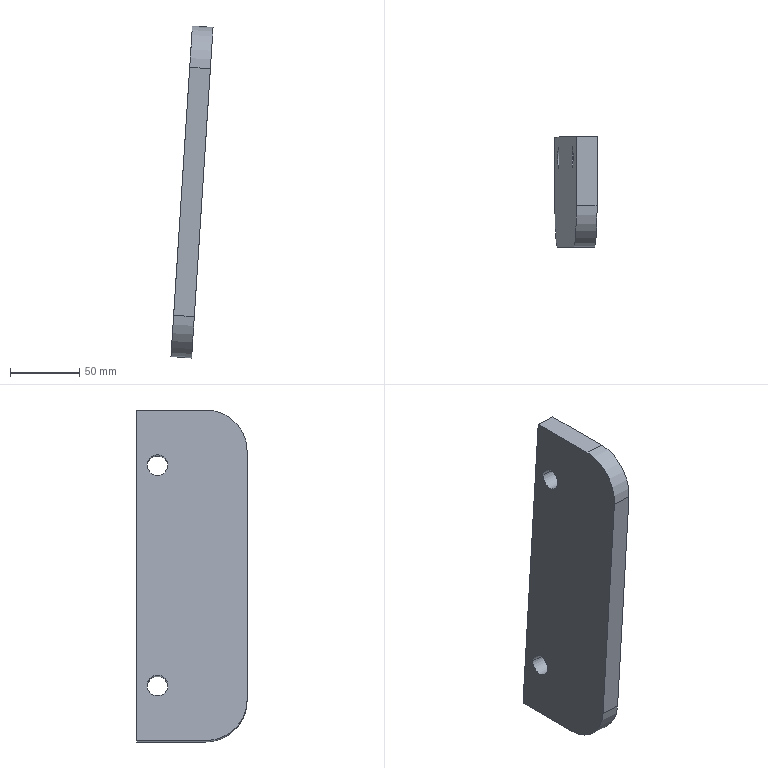Component | SolidWorks | Baffle-2 | 1 solid | 12 faces | box 30.51 x 80 x 240.47 mm | volume 276904 mm3 | cylinder 6 | plane 6 | commonest cylinder face diameters 15 x4 60 x2
build123d program:
from build123d import *

# Parameters (mm, degrees)
BOSS_EXTRUDE1_DEPTH     = 15
CUT_EXTRUDE1_DEPTH      = 697.32
CUT_EXTRUDE1_DEPTH_BACK = 697.32
SKETCH2_R               = 7.5


with BuildPart() as part:
    # Sketch1 → Boss-Extrude1 (new body)
    with BuildSketch(Plane.XY):
        with BuildLine():
            Line((0, 691.546), (50, 691.546))
            ThreePointArc((50, 691.546), (71.213, 682.759), (80, 661.546))
            Line((80, 661.546), (80, 481.546))
            ThreePointArc((80, 481.546), (71.213, 460.333), (50, 451.546))
            Line((50, 451.546), (0, 451.546))
            Line((0, 451.546), (0, 691.546))
        make_face()
    extrude(amount=BOSS_EXTRUDE1_DEPTH)

    # Sketch2 → Cut-Extrude1 (cut, two sides: drawn at the far end of the back side and taken through both)
    with BuildSketch(Plane.XY.offset(15).offset(-CUT_EXTRUDE1_DEPTH_BACK)):
        with Locations((15, 491.546)):
            Circle(SKETCH2_R)
        with Locations((15, 651.546)):
            Circle(SKETCH2_R)
    extrude(amount=CUT_EXTRUDE1_DEPTH + CUT_EXTRUDE1_DEPTH_BACK, mode=Mode.SUBTRACT)


solid = part.part

# Placed as in the assembly
solid = solid.moved(Location((446.042, -801, 253.969), (-180, 86.288, 90)))
STEP:
#1=COLOUR_RGB('',0.7922,0.8196,0.9333);
#2=FILL_AREA_STYLE_COLOUR('',#1);
#3=FILL_AREA_STYLE('',(#2));
#4=SURFACE_STYLE_FILL_AREA(#3);
#5=SURFACE_SIDE_STYLE('',(#4));
#6=SURFACE_STYLE_USAGE(.BOTH.,#5);
#7=PRESENTATION_STYLE_ASSIGNMENT((#6));
#8=CARTESIAN_POINT('',(16.308,-31.831,-9.313));
#9=VERTEX_POINT('',#8);
#10=CARTESIAN_POINT('',(16.308,-32.421,-9.313));
#11=VERTEX_POINT('',#10);
#12=CARTESIAN_POINT('',(16.308,-32.126,-9.313));
#13=DIRECTION('',(0.9979,0.,-0.06474));
#14=DIRECTION('',(0.,-1.,0.));
#15=AXIS2_PLACEMENT_3D('',#12,#13,#14);
#16=CIRCLE('',#15,0.2953);
#17=EDGE_CURVE('',#9,#11,#16,.T.);
#18=ORIENTED_EDGE('',*,*,#17,.F.);
#19=CARTESIAN_POINT('',(16.897,-31.831,-9.351));
#20=VERTEX_POINT('',#19);
#21=CARTESIAN_POINT('',(16.308,-31.831,-9.313));
#22=DIRECTION('',(0.9979,0.,-0.06474));
#23=VECTOR('',#22,39.37);
#24=LINE('',#21,#23);
#25=EDGE_CURVE('',#9,#20,#24,.T.);
#26=ORIENTED_EDGE('',*,*,#25,.T.);
#27=CARTESIAN_POINT('',(16.897,-32.421,-9.351));
#28=VERTEX_POINT('',#27);
#29=CARTESIAN_POINT('',(16.897,-32.126,-9.351));
#30=DIRECTION('',(0.9979,0.,-0.06474));
#31=DIRECTION('',(0.,-1.,0.));
#32=AXIS2_PLACEMENT_3D('',#29,#30,#31);
#33=CIRCLE('',#32,0.2953);
#34=EDGE_CURVE('',#20,#28,#33,.T.);
#35=ORIENTED_EDGE('',*,*,#34,.T.);
#36=CARTESIAN_POINT('',(16.308,-32.421,-9.313));
#37=DIRECTION('',(0.9979,0.,-0.06474));
#38=VECTOR('',#37,39.37);
#39=LINE('',#36,#38);
#40=EDGE_CURVE('',#11,#28,#39,.T.);
#41=ORIENTED_EDGE('',*,*,#40,.F.);
#42=EDGE_LOOP('',(#18,#26,#35,#41));
#43=FACE_OUTER_BOUND('',#42,.T.);
#44=CARTESIAN_POINT('',(16.308,-32.126,-9.313));
#45=DIRECTION('',(0.9979,0.,-0.06474));
#46=DIRECTION('',(0.,-1.,0.));
#47=AXIS2_PLACEMENT_3D('',#44,#45,#46);
#48=CYLINDRICAL_SURFACE('',#47,0.2953);
#49=ADVANCED_FACE('',(#43),#48,.F.);
#50=CARTESIAN_POINT('',(15.9,-31.831,-15.599));
#51=VERTEX_POINT('',#50);
#52=CARTESIAN_POINT('',(15.9,-32.421,-15.599));
#53=VERTEX_POINT('',#52);
#54=CARTESIAN_POINT('',(15.9,-32.126,-15.599));
#55=DIRECTION('',(0.9979,0.,-0.06474));
#56=DIRECTION('',(0.,1.,0.));
#57=AXIS2_PLACEMENT_3D('',#54,#55,#56);
#58=CIRCLE('',#57,0.2953);
#59=EDGE_CURVE('',#51,#53,#58,.T.);
#60=ORIENTED_EDGE('',*,*,#59,.F.);
#61=CARTESIAN_POINT('',(16.489,-31.831,-15.637));
#62=VERTEX_POINT('',#61);
#63=CARTESIAN_POINT('',(15.9,-31.831,-15.599));
#64=DIRECTION('',(0.9979,0.,-0.06474));
#65=VECTOR('',#64,39.37);
#66=LINE('',#63,#65);
#67=EDGE_CURVE('',#51,#62,#66,.T.);
#68=ORIENTED_EDGE('',*,*,#67,.T.);
#69=CARTESIAN_POINT('',(16.489,-32.421,-15.637));
#70=VERTEX_POINT('',#69);
#71=CARTESIAN_POINT('',(16.489,-32.126,-15.637));
#72=DIRECTION('',(0.9979,0.,-0.06474));
#73=DIRECTION('',(0.,-1.,0.));
#74=AXIS2_PLACEMENT_3D('',#71,#72,#73);
#75=CIRCLE('',#74,0.2953);
#76=EDGE_CURVE('',#62,#70,#75,.T.);
#77=ORIENTED_EDGE('',*,*,#76,.T.);
#78=CARTESIAN_POINT('',(15.9,-32.421,-15.599));
#79=DIRECTION('',(0.9979,0.,-0.06474));
#80=VECTOR('',#79,39.37);
#81=LINE('',#78,#80);
#82=EDGE_CURVE('',#53,#70,#81,.T.);
#83=ORIENTED_EDGE('',*,*,#82,.F.);
#84=EDGE_LOOP('',(#60,#68,#77,#83));
#85=FACE_OUTER_BOUND('',#84,.T.);
#86=CARTESIAN_POINT('',(15.9,-32.126,-15.599));
#87=DIRECTION('',(0.9979,0.,-0.06474));
#88=DIRECTION('',(0.,-1.,0.));
#89=AXIS2_PLACEMENT_3D('',#86,#87,#88);
#90=CYLINDRICAL_SURFACE('',#89,0.2953);
#91=ADVANCED_FACE('',(#85),#90,.F.);
#92=CARTESIAN_POINT('',(15.798,-31.535,-17.17));
#93=VERTEX_POINT('',#92);
#94=CARTESIAN_POINT('',(16.41,-31.535,-7.741));
#95=VERTEX_POINT('',#94);
#96=CARTESIAN_POINT('',(15.798,-31.535,-17.17));
#97=DIRECTION('',(0.06474,0.,0.9979));
#98=VECTOR('',#97,39.37);
#99=LINE('',#96,#98);
#100=EDGE_CURVE('',#93,#95,#99,.T.);
#101=ORIENTED_EDGE('',*,*,#100,.T.);
#102=CARTESIAN_POINT('',(16.999,-31.535,-7.78));
#103=VERTEX_POINT('',#102);
#104=CARTESIAN_POINT('',(16.999,-31.535,-7.78));
#105=DIRECTION('',(-0.9979,-0.,0.06474));
#106=VECTOR('',#105,39.37);
#107=LINE('',#104,#106);
#108=EDGE_CURVE('',#103,#95,#107,.T.);
#109=ORIENTED_EDGE('',*,*,#108,.F.);
#110=CARTESIAN_POINT('',(16.387,-31.535,-17.209));
#111=VERTEX_POINT('',#110);
#112=CARTESIAN_POINT('',(16.387,-31.535,-17.209));
#113=DIRECTION('',(0.06474,0.,0.9979));
#114=VECTOR('',#113,39.37);
#115=LINE('',#112,#114);
#116=EDGE_CURVE('',#111,#103,#115,.T.);
#117=ORIENTED_EDGE('',*,*,#116,.F.);
#118=CARTESIAN_POINT('',(16.387,-31.535,-17.209));
#119=DIRECTION('',(-0.9979,-0.,0.06474));
#120=VECTOR('',#119,39.37);
#121=LINE('',#118,#120);
#122=EDGE_CURVE('',#111,#93,#121,.T.);
#123=ORIENTED_EDGE('',*,*,#122,.T.);
#124=EDGE_LOOP('',(#101,#109,#117,#123));
#125=FACE_OUTER_BOUND('',#124,.T.);
#126=CARTESIAN_POINT('',(16.387,-31.535,-17.209));
#127=DIRECTION('',(0.,-1.,-0.));
#128=DIRECTION('',(-0.9979,-0.,0.06474));
#129=AXIS2_PLACEMENT_3D('',#126,#127,#128);
#130=PLANE('',#129);
#131=ADVANCED_FACE('',(#125),#130,.F.);
#132=CARTESIAN_POINT('',(16.41,-33.504,-7.741));
#133=VERTEX_POINT('',#132);
#134=CARTESIAN_POINT('',(16.41,-31.535,-7.741));
#135=DIRECTION('',(0.,-1.,-0.));
#136=VECTOR('',#135,39.37);
#137=LINE('',#134,#136);
#138=EDGE_CURVE('',#95,#133,#137,.T.);
#139=ORIENTED_EDGE('',*,*,#138,.T.);
#140=CARTESIAN_POINT('',(16.999,-33.504,-7.78));
#141=VERTEX_POINT('',#140);
#142=CARTESIAN_POINT('',(16.999,-33.504,-7.78));
#143=DIRECTION('',(-0.9979,-0.,0.06474));
#144=VECTOR('',#143,39.37);
#145=LINE('',#142,#144);
#146=EDGE_CURVE('',#141,#133,#145,.T.);
#147=ORIENTED_EDGE('',*,*,#146,.F.);
#148=CARTESIAN_POINT('',(16.999,-31.535,-7.78));
#149=DIRECTION('',(0.,-1.,-0.));
#150=VECTOR('',#149,39.37);
#151=LINE('',#148,#150);
#152=EDGE_CURVE('',#103,#141,#151,.T.);
#153=ORIENTED_EDGE('',*,*,#152,.F.);
#154=ORIENTED_EDGE('',*,*,#108,.T.);
#155=EDGE_LOOP('',(#139,#147,#153,#154));
#156=FACE_OUTER_BOUND('',#155,.T.);
#157=CARTESIAN_POINT('',(16.999,-31.535,-7.78));
#158=DIRECTION('',(-0.06474,-0.,-0.9979));
#159=DIRECTION('',(0.9979,0.,-0.06474));
#160=AXIS2_PLACEMENT_3D('',#157,#158,#159);
#161=PLANE('',#160);
#162=ADVANCED_FACE('',(#156),#161,.F.);
#163=CARTESIAN_POINT('',(16.333,-34.685,-8.92));
#164=VERTEX_POINT('',#163);
#165=CARTESIAN_POINT('',(16.333,-33.504,-8.92));
#166=DIRECTION('',(0.9979,0.,-0.06474));
#167=DIRECTION('',(0.,-1.,0.));
#168=AXIS2_PLACEMENT_3D('',#165,#166,#167);
#169=CIRCLE('',#168,1.181);
#170=EDGE_CURVE('',#133,#164,#169,.T.);
#171=ORIENTED_EDGE('',*,*,#170,.T.);
#172=CARTESIAN_POINT('',(16.923,-34.685,-8.958));
#173=VERTEX_POINT('',#172);
#174=CARTESIAN_POINT('',(16.923,-34.685,-8.958));
#175=DIRECTION('',(-0.9979,-0.,0.06474));
#176=VECTOR('',#175,39.37);
#177=LINE('',#174,#176);
#178=EDGE_CURVE('',#173,#164,#177,.T.);
#179=ORIENTED_EDGE('',*,*,#178,.F.);
#180=CARTESIAN_POINT('',(16.923,-33.504,-8.958));
#181=DIRECTION('',(0.9979,0.,-0.06474));
#182=DIRECTION('',(0.,-1.,0.));
#183=AXIS2_PLACEMENT_3D('',#180,#181,#182);
#184=CIRCLE('',#183,1.181);
#185=EDGE_CURVE('',#141,#173,#184,.T.);
#186=ORIENTED_EDGE('',*,*,#185,.F.);
#187=ORIENTED_EDGE('',*,*,#146,.T.);
#188=EDGE_LOOP('',(#171,#179,#186,#187));
#189=FACE_OUTER_BOUND('',#188,.T.);
#190=CARTESIAN_POINT('',(16.923,-33.504,-8.958));
#191=DIRECTION('',(-0.9979,-0.,0.06474));
#192=DIRECTION('',(0.,1.,0.));
#193=AXIS2_PLACEMENT_3D('',#190,#191,#192);
#194=CYLINDRICAL_SURFACE('',#193,1.181);
#195=ADVANCED_FACE('',(#189),#194,.T.);
#196=CARTESIAN_POINT('',(15.875,-34.685,-15.992));
#197=VERTEX_POINT('',#196);
#198=CARTESIAN_POINT('',(15.875,-34.685,-15.992));
#199=DIRECTION('',(-0.06474,0.,-0.9979));
#200=VECTOR('',#199,39.37);
#201=LINE('',#198,#200);
#202=EDGE_CURVE('',#164,#197,#201,.T.);
#203=ORIENTED_EDGE('',*,*,#202,.T.);
#204=CARTESIAN_POINT('',(16.464,-34.685,-16.03));
#205=VERTEX_POINT('',#204);
#206=CARTESIAN_POINT('',(16.464,-34.685,-16.03));
#207=DIRECTION('',(-0.9979,-0.,0.06474));
#208=VECTOR('',#207,39.37);
#209=LINE('',#206,#208);
#210=EDGE_CURVE('',#205,#197,#209,.T.);
#211=ORIENTED_EDGE('',*,*,#210,.F.);
#212=CARTESIAN_POINT('',(16.464,-34.685,-16.03));
#213=DIRECTION('',(-0.06474,0.,-0.9979));
#214=VECTOR('',#213,39.37);
#215=LINE('',#212,#214);
#216=EDGE_CURVE('',#173,#205,#215,.T.);
#217=ORIENTED_EDGE('',*,*,#216,.F.);
#218=ORIENTED_EDGE('',*,*,#178,.T.);
#219=EDGE_LOOP('',(#203,#211,#217,#218));
#220=FACE_OUTER_BOUND('',#219,.T.);
#221=CARTESIAN_POINT('',(16.464,-34.685,-16.03));
#222=DIRECTION('',(-0.,1.,0.));
#223=DIRECTION('',(0.06474,-0.,0.9979));
#224=AXIS2_PLACEMENT_3D('',#221,#222,#223);
#225=PLANE('',#224);
#226=ADVANCED_FACE('',(#220),#225,.F.);
#227=CARTESIAN_POINT('',(15.798,-33.504,-17.17));
#228=VERTEX_POINT('',#227);
#229=CARTESIAN_POINT('',(15.875,-33.504,-15.992));
#230=DIRECTION('',(0.9979,0.,-0.06474));
#231=DIRECTION('',(0.,1.,0.));
#232=AXIS2_PLACEMENT_3D('',#229,#230,#231);
#233=CIRCLE('',#232,1.181);
#234=EDGE_CURVE('',#197,#228,#233,.T.);
#235=ORIENTED_EDGE('',*,*,#234,.T.);
#236=CARTESIAN_POINT('',(16.387,-33.504,-17.209));
#237=VERTEX_POINT('',#236);
#238=CARTESIAN_POINT('',(16.387,-33.504,-17.209));
#239=DIRECTION('',(-0.9979,-0.,0.06474));
#240=VECTOR('',#239,39.37);
#241=LINE('',#238,#240);
#242=EDGE_CURVE('',#237,#228,#241,.T.);
#243=ORIENTED_EDGE('',*,*,#242,.F.);
#244=CARTESIAN_POINT('',(16.464,-33.504,-16.03));
#245=DIRECTION('',(0.9979,0.,-0.06474));
#246=DIRECTION('',(0.,1.,0.));
#247=AXIS2_PLACEMENT_3D('',#244,#245,#246);
#248=CIRCLE('',#247,1.181);
#249=EDGE_CURVE('',#205,#237,#248,.T.);
#250=ORIENTED_EDGE('',*,*,#249,.F.);
#251=ORIENTED_EDGE('',*,*,#210,.T.);
#252=EDGE_LOOP('',(#235,#243,#250,#251));
#253=FACE_OUTER_BOUND('',#252,.T.);
#254=CARTESIAN_POINT('',(16.464,-33.504,-16.03));
#255=DIRECTION('',(-0.9979,-0.,0.06474));
#256=DIRECTION('',(0.,1.,0.));
#257=AXIS2_PLACEMENT_3D('',#254,#255,#256);
#258=CYLINDRICAL_SURFACE('',#257,1.181);
#259=ADVANCED_FACE('',(#253),#258,.T.);
#260=CARTESIAN_POINT('',(15.798,-31.535,-17.17));
#261=DIRECTION('',(-0.,1.,0.));
#262=VECTOR('',#261,39.37);
#263=LINE('',#260,#262);
#264=EDGE_CURVE('',#228,#93,#263,.T.);
#265=ORIENTED_EDGE('',*,*,#264,.T.);
#266=ORIENTED_EDGE('',*,*,#122,.F.);
#267=CARTESIAN_POINT('',(16.387,-31.535,-17.209));
#268=DIRECTION('',(-0.,1.,0.));
#269=VECTOR('',#268,39.37);
#270=LINE('',#267,#269);
#271=EDGE_CURVE('',#237,#111,#270,.T.);
#272=ORIENTED_EDGE('',*,*,#271,.F.);
#273=ORIENTED_EDGE('',*,*,#242,.T.);
#274=EDGE_LOOP('',(#265,#266,#272,#273));
#275=FACE_OUTER_BOUND('',#274,.T.);
#276=CARTESIAN_POINT('',(16.387,-31.535,-17.209));
#277=DIRECTION('',(0.06474,0.,0.9979));
#278=DIRECTION('',(-0.9979,-0.,0.06474));
#279=AXIS2_PLACEMENT_3D('',#276,#277,#278);
#280=PLANE('',#279);
#281=ADVANCED_FACE('',(#275),#280,.F.);
#282=CARTESIAN_POINT('',(16.897,-32.126,-9.351));
#283=DIRECTION('',(0.9979,0.,-0.06474));
#284=DIRECTION('',(0.,-1.,0.));
#285=AXIS2_PLACEMENT_3D('',#282,#283,#284);
#286=CIRCLE('',#285,0.2953);
#287=EDGE_CURVE('',#28,#20,#286,.T.);
#288=ORIENTED_EDGE('',*,*,#287,.F.);
#289=ORIENTED_EDGE('',*,*,#34,.F.);
#290=EDGE_LOOP('',(#288,#289));
#291=FACE_BOUND('',#290,.T.);
#292=CARTESIAN_POINT('',(16.489,-32.126,-15.637));
#293=DIRECTION('',(0.9979,0.,-0.06474));
#294=DIRECTION('',(0.,-1.,0.));
#295=AXIS2_PLACEMENT_3D('',#292,#293,#294);
#296=CIRCLE('',#295,0.2953);
#297=EDGE_CURVE('',#70,#62,#296,.T.);
#298=ORIENTED_EDGE('',*,*,#297,.F.);
#299=ORIENTED_EDGE('',*,*,#76,.F.);
#300=EDGE_LOOP('',(#298,#299));
#301=FACE_BOUND('',#300,.T.);
#302=ORIENTED_EDGE('',*,*,#116,.T.);
#303=ORIENTED_EDGE('',*,*,#152,.T.);
#304=ORIENTED_EDGE('',*,*,#185,.T.);
#305=ORIENTED_EDGE('',*,*,#216,.T.);
#306=ORIENTED_EDGE('',*,*,#249,.T.);
#307=ORIENTED_EDGE('',*,*,#271,.T.);
#308=EDGE_LOOP('',(#302,#303,#304,#305,#306,#307));
#309=FACE_OUTER_BOUND('',#308,.T.);
#310=CARTESIAN_POINT('',(16.923,-33.504,-8.958));
#311=DIRECTION('',(0.9979,0.,-0.06474));
#312=DIRECTION('',(0.,-1.,-0.));
#313=AXIS2_PLACEMENT_3D('',#310,#311,#312);
#314=PLANE('',#313);
#315=ADVANCED_FACE('',(#291,#301,#309),#314,.T.);
#316=CARTESIAN_POINT('',(16.308,-32.126,-9.313));
#317=DIRECTION('',(0.9979,0.,-0.06474));
#318=DIRECTION('',(0.,-1.,0.));
#319=AXIS2_PLACEMENT_3D('',#316,#317,#318);
#320=CIRCLE('',#319,0.2953);
#321=EDGE_CURVE('',#11,#9,#320,.T.);
#322=ORIENTED_EDGE('',*,*,#321,.T.);
#323=ORIENTED_EDGE('',*,*,#17,.T.);
#324=EDGE_LOOP('',(#322,#323));
#325=FACE_BOUND('',#324,.T.);
#326=CARTESIAN_POINT('',(15.9,-32.126,-15.599));
#327=DIRECTION('',(0.9979,0.,-0.06474));
#328=DIRECTION('',(0.,1.,0.));
#329=AXIS2_PLACEMENT_3D('',#326,#327,#328);
#330=CIRCLE('',#329,0.2953);
#331=EDGE_CURVE('',#53,#51,#330,.T.);
#332=ORIENTED_EDGE('',*,*,#331,.T.);
#333=ORIENTED_EDGE('',*,*,#59,.T.);
#334=EDGE_LOOP('',(#332,#333));
#335=FACE_BOUND('',#334,.T.);
#336=ORIENTED_EDGE('',*,*,#100,.F.);
#337=ORIENTED_EDGE('',*,*,#264,.F.);
#338=ORIENTED_EDGE('',*,*,#234,.F.);
#339=ORIENTED_EDGE('',*,*,#202,.F.);
#340=ORIENTED_EDGE('',*,*,#170,.F.);
#341=ORIENTED_EDGE('',*,*,#138,.F.);
#342=EDGE_LOOP('',(#336,#337,#338,#339,#340,#341));
#343=FACE_OUTER_BOUND('',#342,.T.);
#344=CARTESIAN_POINT('',(16.333,-33.504,-8.92));
#345=DIRECTION('',(0.9979,0.,-0.06474));
#346=DIRECTION('',(0.,-1.,-0.));
#347=AXIS2_PLACEMENT_3D('',#344,#345,#346);
#348=PLANE('',#347);
#349=ADVANCED_FACE('',(#325,#335,#343),#348,.F.);
#350=ORIENTED_EDGE('',*,*,#67,.F.);
#351=ORIENTED_EDGE('',*,*,#331,.F.);
#352=ORIENTED_EDGE('',*,*,#82,.T.);
#353=ORIENTED_EDGE('',*,*,#297,.T.);
#354=EDGE_LOOP('',(#350,#351,#352,#353));
#355=FACE_OUTER_BOUND('',#354,.T.);
#356=CARTESIAN_POINT('',(15.9,-32.126,-15.599));
#357=DIRECTION('',(0.9979,0.,-0.06474));
#358=DIRECTION('',(0.,-1.,0.));
#359=AXIS2_PLACEMENT_3D('',#356,#357,#358);
#360=CYLINDRICAL_SURFACE('',#359,0.2953);
#361=ADVANCED_FACE('',(#355),#360,.F.);
#362=ORIENTED_EDGE('',*,*,#25,.F.);
#363=ORIENTED_EDGE('',*,*,#321,.F.);
#364=ORIENTED_EDGE('',*,*,#40,.T.);
#365=ORIENTED_EDGE('',*,*,#287,.T.);
#366=EDGE_LOOP('',(#362,#363,#364,#365));
#367=FACE_OUTER_BOUND('',#366,.T.);
#368=CARTESIAN_POINT('',(16.308,-32.126,-9.313));
#369=DIRECTION('',(0.9979,0.,-0.06474));
#370=DIRECTION('',(0.,-1.,0.));
#371=AXIS2_PLACEMENT_3D('',#368,#369,#370);
#372=CYLINDRICAL_SURFACE('',#371,0.2953);
#373=ADVANCED_FACE('',(#367),#372,.F.);
#374=CLOSED_SHELL('',(#49,#91,#131,#162,#195,#226,#259,#281,#315,#349,#361,#373));
#375=MANIFOLD_SOLID_BREP('',#374);
#376=STYLED_ITEM('',(#7),#375);
#377=(LENGTH_UNIT()NAMED_UNIT(*)SI_UNIT($,.METRE.));
#378=LENGTH_MEASURE_WITH_UNIT(LENGTH_MEASURE(0.0254),#377);
#379=DIMENSIONAL_EXPONENTS(1.,0.,0.,0.,0.,0.,0.);
#380=(CONVERSION_BASED_UNIT('',#378)LENGTH_UNIT()NAMED_UNIT(#379));
#381=UNCERTAINTY_MEASURE_WITH_UNIT(LENGTH_MEASURE(0.00001),#380,'','');
#382=(NAMED_UNIT(*)PLANE_ANGLE_UNIT()SI_UNIT($,.RADIAN.));
#383=(NAMED_UNIT(*)SI_UNIT($,.STERADIAN.)SOLID_ANGLE_UNIT());
#384=(GEOMETRIC_REPRESENTATION_CONTEXT(3)GLOBAL_UNCERTAINTY_ASSIGNED_CONTEXT((#381))GLOBAL_UNIT_ASSIGNED_CONTEXT((#380,#382,#383))REPRESENTATION_CONTEXT('',''));
#385=MECHANICAL_DESIGN_GEOMETRIC_PRESENTATION_REPRESENTATION('',(#376),#384);
#386=CARTESIAN_POINT('',(0.,0.,0.));
#387=DIRECTION('',(0.,0.,1.));
#388=DIRECTION('',(1.,0.,0.));
#389=AXIS2_PLACEMENT_3D('',#386,#387,#388);
#390=(LENGTH_UNIT()NAMED_UNIT(*)SI_UNIT($,.METRE.));
#391=LENGTH_MEASURE_WITH_UNIT(LENGTH_MEASURE(0.0254),#390);
#392=DIMENSIONAL_EXPONENTS(1.,0.,0.,0.,0.,0.,0.);
#393=(CONVERSION_BASED_UNIT('',#391)LENGTH_UNIT()NAMED_UNIT(#392));
#394=UNCERTAINTY_MEASURE_WITH_UNIT(LENGTH_MEASURE(0.00001),#393,'','');
#395=(NAMED_UNIT(*)PLANE_ANGLE_UNIT()SI_UNIT($,.RADIAN.));
#396=(NAMED_UNIT(*)SI_UNIT($,.STERADIAN.)SOLID_ANGLE_UNIT());
#397=(GEOMETRIC_REPRESENTATION_CONTEXT(3)GLOBAL_UNCERTAINTY_ASSIGNED_CONTEXT((#394))GLOBAL_UNIT_ASSIGNED_CONTEXT((#393,#395,#396))REPRESENTATION_CONTEXT('',''));
#398=ADVANCED_BREP_SHAPE_REPRESENTATION('',(#375,#389),#397);
#399=PRESENTATION_LAYER_ASSIGNMENT('','',(#376));